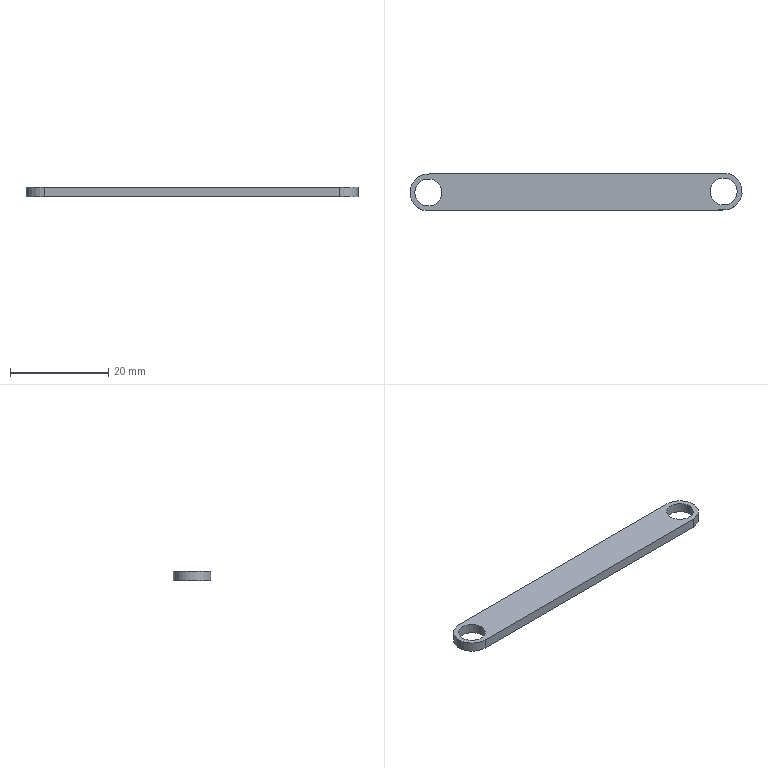Component | NX | CRANK_ROCKER_1 | 1 solid | 8 faces | box 67.5 x 7.69 x 2 mm | volume 893 mm3 | cylinder 4 | plane 4 | commonest cylinder face diameters 7.5 x2 5.5 x2
STEP:
#1=CARTESIAN_POINT('',(0.,0.,0.));
#2=DIRECTION('',(0.,0.,1.));
#3=DIRECTION('',(1.,0.,0.));
#4=AXIS2_PLACEMENT_3D('',#1,#2,#3);
#5=CARTESIAN_POINT('',(-30.015,-12.024,-10.49));
#6=VERTEX_POINT('',#5);
#7=CARTESIAN_POINT('',(-29.991,-19.524,-10.49));
#8=VERTEX_POINT('',#7);
#9=CARTESIAN_POINT('',(-30.003,-15.774,-10.49));
#10=DIRECTION('',(0.,0.,1.));
#11=DIRECTION('',(1.,0.003165,0.));
#12=AXIS2_PLACEMENT_3D('',#9,#10,#11);
#13=CIRCLE('',#12,3.75);
#14=CARTESIAN_POINT('',(-30.003,-15.774,-8.49));
#15=DIRECTION('',(0.,0.,-1.));
#16=DIRECTION('',(-1.,-0.003165,0.));
#17=AXIS2_PLACEMENT_3D('',#14,#15,#16);
#18=CYLINDRICAL_SURFACE('',#17,3.75);
#19=CARTESIAN_POINT('',(9.425,2.));
#20=DIRECTION('',(-1.,0.));
#21=VECTOR('',#20,1.);
#22=LINE('',#19,#21);
#23=(GEOMETRIC_REPRESENTATION_CONTEXT(2)PARAMETRIC_REPRESENTATION_CONTEXT()REPRESENTATION_CONTEXT('',''));
#24=DEFINITIONAL_REPRESENTATION('',(#22),#23);
#25=PCURVE('',#18,#24);
#26=CARTESIAN_POINT('',(-30.003,-15.774,-10.49));
#27=DIRECTION('',(0.,0.,1.));
#28=DIRECTION('',(1.,0.003165,0.));
#29=AXIS2_PLACEMENT_3D('',#26,#27,#28);
#30=PLANE('',#29);
#31=CARTESIAN_POINT('',(0.,0.));
#32=DIRECTION('',(1.,-0.));
#33=AXIS2_PLACEMENT_2D('',#31,#32);
#34=CIRCLE('',#33,3.75);
#35=(GEOMETRIC_REPRESENTATION_CONTEXT(2)PARAMETRIC_REPRESENTATION_CONTEXT()REPRESENTATION_CONTEXT('',''));
#36=DEFINITIONAL_REPRESENTATION('',(#34),#35);
#37=PCURVE('',#30,#36);
#38=SURFACE_CURVE('',#13,(#25,#37),.PCURVE_S1.);
#39=EDGE_CURVE('',#6,#8,#38,.T.);
#40=ORIENTED_EDGE('',*,*,#39,.T.);
#41=CARTESIAN_POINT('',(-29.991,-19.524,-8.49));
#42=VERTEX_POINT('',#41);
#43=CARTESIAN_POINT('',(-29.991,-19.524,-8.49));
#44=DIRECTION('',(0.,0.,-1.));
#45=VECTOR('',#44,1.);
#46=LINE('',#43,#45);
#47=CARTESIAN_POINT('',(4.712,0.));
#48=DIRECTION('',(0.,1.));
#49=VECTOR('',#48,1.);
#50=LINE('',#47,#49);
#51=(GEOMETRIC_REPRESENTATION_CONTEXT(2)PARAMETRIC_REPRESENTATION_CONTEXT()REPRESENTATION_CONTEXT('',''));
#52=DEFINITIONAL_REPRESENTATION('',(#50),#51);
#53=PCURVE('',#18,#52);
#54=CARTESIAN_POINT('',(-29.991,-19.524,-8.49));
#55=DIRECTION('',(-0.003165,1.,0.));
#56=DIRECTION('',(-1.,-0.003165,0.));
#57=AXIS2_PLACEMENT_3D('',#54,#55,#56);
#58=PLANE('',#57);
#59=CARTESIAN_POINT('',(-0.,0.));
#60=DIRECTION('',(0.,-1.));
#61=VECTOR('',#60,1.);
#62=LINE('',#59,#61);
#63=(GEOMETRIC_REPRESENTATION_CONTEXT(2)PARAMETRIC_REPRESENTATION_CONTEXT()REPRESENTATION_CONTEXT('',''));
#64=DEFINITIONAL_REPRESENTATION('',(#62),#63);
#65=PCURVE('',#58,#64);
#66=SURFACE_CURVE('',#46,(#53,#65),.PCURVE_S1.);
#67=EDGE_CURVE('',#42,#8,#66,.T.);
#68=ORIENTED_EDGE('',*,*,#67,.F.);
#69=CARTESIAN_POINT('',(-30.015,-12.024,-8.49));
#70=VERTEX_POINT('',#69);
#71=CARTESIAN_POINT('',(-30.003,-15.774,-8.49));
#72=DIRECTION('',(0.,0.,1.));
#73=DIRECTION('',(1.,0.003165,0.));
#74=AXIS2_PLACEMENT_3D('',#71,#72,#73);
#75=CIRCLE('',#74,3.75);
#76=CARTESIAN_POINT('',(9.425,0.));
#77=DIRECTION('',(-1.,0.));
#78=VECTOR('',#77,1.);
#79=LINE('',#76,#78);
#80=(GEOMETRIC_REPRESENTATION_CONTEXT(2)PARAMETRIC_REPRESENTATION_CONTEXT()REPRESENTATION_CONTEXT('',''));
#81=DEFINITIONAL_REPRESENTATION('',(#79),#80);
#82=PCURVE('',#18,#81);
#83=CARTESIAN_POINT('',(-30.003,-15.774,-8.49));
#84=DIRECTION('',(0.,0.,1.));
#85=DIRECTION('',(1.,0.003165,0.));
#86=AXIS2_PLACEMENT_3D('',#83,#84,#85);
#87=PLANE('',#86);
#88=CARTESIAN_POINT('',(0.,0.));
#89=DIRECTION('',(1.,-0.));
#90=AXIS2_PLACEMENT_2D('',#88,#89);
#91=CIRCLE('',#90,3.75);
#92=(GEOMETRIC_REPRESENTATION_CONTEXT(2)PARAMETRIC_REPRESENTATION_CONTEXT()REPRESENTATION_CONTEXT('',''));
#93=DEFINITIONAL_REPRESENTATION('',(#91),#92);
#94=PCURVE('',#87,#93);
#95=SURFACE_CURVE('',#75,(#82,#94),.PCURVE_S1.);
#96=EDGE_CURVE('',#70,#42,#95,.T.);
#97=ORIENTED_EDGE('',*,*,#96,.F.);
#98=CARTESIAN_POINT('',(-30.015,-12.024,-8.49));
#99=DIRECTION('',(0.,0.,-1.));
#100=VECTOR('',#99,1.);
#101=LINE('',#98,#100);
#102=CARTESIAN_POINT('',(7.854,0.));
#103=DIRECTION('',(0.,1.));
#104=VECTOR('',#103,1.);
#105=LINE('',#102,#104);
#106=(GEOMETRIC_REPRESENTATION_CONTEXT(2)PARAMETRIC_REPRESENTATION_CONTEXT()REPRESENTATION_CONTEXT('',''));
#107=DEFINITIONAL_REPRESENTATION('',(#105),#106);
#108=PCURVE('',#18,#107);
#109=CARTESIAN_POINT('',(29.985,-11.835,-8.49));
#110=DIRECTION('',(0.003165,-1.,0.));
#111=DIRECTION('',(0.,0.,-1.));
#112=AXIS2_PLACEMENT_3D('',#109,#110,#111);
#113=PLANE('',#112);
#114=CARTESIAN_POINT('',(0.,-60.));
#115=DIRECTION('',(1.,0.));
#116=VECTOR('',#115,1.);
#117=LINE('',#114,#116);
#118=(GEOMETRIC_REPRESENTATION_CONTEXT(2)PARAMETRIC_REPRESENTATION_CONTEXT()REPRESENTATION_CONTEXT('',''));
#119=DEFINITIONAL_REPRESENTATION('',(#117),#118);
#120=PCURVE('',#113,#119);
#121=SURFACE_CURVE('',#101,(#108,#120),.PCURVE_S1.);
#122=EDGE_CURVE('',#70,#6,#121,.T.);
#123=ORIENTED_EDGE('',*,*,#122,.T.);
#124=EDGE_LOOP('',(#40,#68,#97,#123));
#125=FACE_BOUND('',#124,.T.);
#126=ADVANCED_FACE('',(#125),#18,.T.);
#127=CARTESIAN_POINT('',(30.008,-19.335,-10.49));
#128=VERTEX_POINT('',#127);
#129=CARTESIAN_POINT('',(-29.991,-19.524,-10.49));
#130=DIRECTION('',(1.,0.003165,0.));
#131=VECTOR('',#130,1.);
#132=LINE('',#129,#131);
#133=CARTESIAN_POINT('',(0.,-2.));
#134=DIRECTION('',(-1.,0.));
#135=VECTOR('',#134,1.);
#136=LINE('',#133,#135);
#137=(GEOMETRIC_REPRESENTATION_CONTEXT(2)PARAMETRIC_REPRESENTATION_CONTEXT()REPRESENTATION_CONTEXT('',''));
#138=DEFINITIONAL_REPRESENTATION('',(#136),#137);
#139=PCURVE('',#58,#138);
#140=CARTESIAN_POINT('',(0.,-3.75));
#141=DIRECTION('',(1.,-0.));
#142=VECTOR('',#141,1.);
#143=LINE('',#140,#142);
#144=(GEOMETRIC_REPRESENTATION_CONTEXT(2)PARAMETRIC_REPRESENTATION_CONTEXT()REPRESENTATION_CONTEXT('',''));
#145=DEFINITIONAL_REPRESENTATION('',(#143),#144);
#146=PCURVE('',#30,#145);
#147=SURFACE_CURVE('',#132,(#139,#146),.PCURVE_S1.);
#148=EDGE_CURVE('',#8,#128,#147,.T.);
#149=ORIENTED_EDGE('',*,*,#148,.T.);
#150=CARTESIAN_POINT('',(30.008,-19.335,-8.49));
#151=VERTEX_POINT('',#150);
#152=CARTESIAN_POINT('',(30.008,-19.335,-8.49));
#153=DIRECTION('',(0.,0.,-1.));
#154=VECTOR('',#153,1.);
#155=LINE('',#152,#154);
#156=CARTESIAN_POINT('',(-60.,0.));
#157=DIRECTION('',(0.,-1.));
#158=VECTOR('',#157,1.);
#159=LINE('',#156,#158);
#160=(GEOMETRIC_REPRESENTATION_CONTEXT(2)PARAMETRIC_REPRESENTATION_CONTEXT()REPRESENTATION_CONTEXT('',''));
#161=DEFINITIONAL_REPRESENTATION('',(#159),#160);
#162=PCURVE('',#58,#161);
#163=CARTESIAN_POINT('',(29.996,-15.585,-8.49));
#164=DIRECTION('',(0.,0.,-1.));
#165=DIRECTION('',(-1.,-0.003165,0.));
#166=AXIS2_PLACEMENT_3D('',#163,#164,#165);
#167=CYLINDRICAL_SURFACE('',#166,3.75);
#168=CARTESIAN_POINT('',(4.712,0.));
#169=DIRECTION('',(0.,1.));
#170=VECTOR('',#169,1.);
#171=LINE('',#168,#170);
#172=(GEOMETRIC_REPRESENTATION_CONTEXT(2)PARAMETRIC_REPRESENTATION_CONTEXT()REPRESENTATION_CONTEXT('',''));
#173=DEFINITIONAL_REPRESENTATION('',(#171),#172);
#174=PCURVE('',#167,#173);
#175=SURFACE_CURVE('',#155,(#162,#174),.PCURVE_S1.);
#176=EDGE_CURVE('',#151,#128,#175,.T.);
#177=ORIENTED_EDGE('',*,*,#176,.F.);
#178=CARTESIAN_POINT('',(-29.991,-19.524,-8.49));
#179=DIRECTION('',(1.,0.003165,0.));
#180=VECTOR('',#179,1.);
#181=LINE('',#178,#180);
#182=CARTESIAN_POINT('',(0.,0.));
#183=DIRECTION('',(-1.,0.));
#184=VECTOR('',#183,1.);
#185=LINE('',#182,#184);
#186=(GEOMETRIC_REPRESENTATION_CONTEXT(2)PARAMETRIC_REPRESENTATION_CONTEXT()REPRESENTATION_CONTEXT('',''));
#187=DEFINITIONAL_REPRESENTATION('',(#185),#186);
#188=PCURVE('',#58,#187);
#189=CARTESIAN_POINT('',(0.,-3.75));
#190=DIRECTION('',(1.,-0.));
#191=VECTOR('',#190,1.);
#192=LINE('',#189,#191);
#193=(GEOMETRIC_REPRESENTATION_CONTEXT(2)PARAMETRIC_REPRESENTATION_CONTEXT()REPRESENTATION_CONTEXT('',''));
#194=DEFINITIONAL_REPRESENTATION('',(#192),#193);
#195=PCURVE('',#87,#194);
#196=SURFACE_CURVE('',#181,(#188,#195),.PCURVE_S1.);
#197=EDGE_CURVE('',#42,#151,#196,.T.);
#198=ORIENTED_EDGE('',*,*,#197,.F.);
#199=ORIENTED_EDGE('',*,*,#67,.T.);
#200=EDGE_LOOP('',(#149,#177,#198,#199));
#201=FACE_BOUND('',#200,.T.);
#202=ADVANCED_FACE('',(#201),#58,.F.);
#203=CARTESIAN_POINT('',(29.985,-11.835,-10.49));
#204=VERTEX_POINT('',#203);
#205=CARTESIAN_POINT('',(29.996,-15.585,-10.49));
#206=DIRECTION('',(0.,0.,1.));
#207=DIRECTION('',(1.,0.003165,0.));
#208=AXIS2_PLACEMENT_3D('',#205,#206,#207);
#209=CIRCLE('',#208,3.75);
#210=CARTESIAN_POINT('',(9.425,2.));
#211=DIRECTION('',(-1.,0.));
#212=VECTOR('',#211,1.);
#213=LINE('',#210,#212);
#214=(GEOMETRIC_REPRESENTATION_CONTEXT(2)PARAMETRIC_REPRESENTATION_CONTEXT()REPRESENTATION_CONTEXT('',''));
#215=DEFINITIONAL_REPRESENTATION('',(#213),#214);
#216=PCURVE('',#167,#215);
#217=CARTESIAN_POINT('',(60.,-0.));
#218=DIRECTION('',(1.,-0.));
#219=AXIS2_PLACEMENT_2D('',#217,#218);
#220=CIRCLE('',#219,3.75);
#221=(GEOMETRIC_REPRESENTATION_CONTEXT(2)PARAMETRIC_REPRESENTATION_CONTEXT()REPRESENTATION_CONTEXT('',''));
#222=DEFINITIONAL_REPRESENTATION('',(#220),#221);
#223=PCURVE('',#30,#222);
#224=SURFACE_CURVE('',#209,(#216,#223),.PCURVE_S1.);
#225=EDGE_CURVE('',#128,#204,#224,.T.);
#226=ORIENTED_EDGE('',*,*,#225,.T.);
#227=CARTESIAN_POINT('',(29.985,-11.835,-8.49));
#228=VERTEX_POINT('',#227);
#229=CARTESIAN_POINT('',(29.985,-11.835,-8.49));
#230=DIRECTION('',(0.,0.,-1.));
#231=VECTOR('',#230,1.);
#232=LINE('',#229,#231);
#233=CARTESIAN_POINT('',(1.571,0.));
#234=DIRECTION('',(0.,1.));
#235=VECTOR('',#234,1.);
#236=LINE('',#233,#235);
#237=(GEOMETRIC_REPRESENTATION_CONTEXT(2)PARAMETRIC_REPRESENTATION_CONTEXT()REPRESENTATION_CONTEXT('',''));
#238=DEFINITIONAL_REPRESENTATION('',(#236),#237);
#239=PCURVE('',#167,#238);
#240=CARTESIAN_POINT('',(0.,0.));
#241=DIRECTION('',(1.,0.));
#242=VECTOR('',#241,1.);
#243=LINE('',#240,#242);
#244=(GEOMETRIC_REPRESENTATION_CONTEXT(2)PARAMETRIC_REPRESENTATION_CONTEXT()REPRESENTATION_CONTEXT('',''));
#245=DEFINITIONAL_REPRESENTATION('',(#243),#244);
#246=PCURVE('',#113,#245);
#247=SURFACE_CURVE('',#232,(#239,#246),.PCURVE_S1.);
#248=EDGE_CURVE('',#228,#204,#247,.T.);
#249=ORIENTED_EDGE('',*,*,#248,.F.);
#250=CARTESIAN_POINT('',(29.996,-15.585,-8.49));
#251=DIRECTION('',(0.,0.,1.));
#252=DIRECTION('',(1.,0.003165,0.));
#253=AXIS2_PLACEMENT_3D('',#250,#251,#252);
#254=CIRCLE('',#253,3.75);
#255=CARTESIAN_POINT('',(9.425,0.));
#256=DIRECTION('',(-1.,0.));
#257=VECTOR('',#256,1.);
#258=LINE('',#255,#257);
#259=(GEOMETRIC_REPRESENTATION_CONTEXT(2)PARAMETRIC_REPRESENTATION_CONTEXT()REPRESENTATION_CONTEXT('',''));
#260=DEFINITIONAL_REPRESENTATION('',(#258),#259);
#261=PCURVE('',#167,#260);
#262=CARTESIAN_POINT('',(60.,-0.));
#263=DIRECTION('',(1.,-0.));
#264=AXIS2_PLACEMENT_2D('',#262,#263);
#265=CIRCLE('',#264,3.75);
#266=(GEOMETRIC_REPRESENTATION_CONTEXT(2)PARAMETRIC_REPRESENTATION_CONTEXT()REPRESENTATION_CONTEXT('',''));
#267=DEFINITIONAL_REPRESENTATION('',(#265),#266);
#268=PCURVE('',#87,#267);
#269=SURFACE_CURVE('',#254,(#261,#268),.PCURVE_S1.);
#270=EDGE_CURVE('',#151,#228,#269,.T.);
#271=ORIENTED_EDGE('',*,*,#270,.F.);
#272=ORIENTED_EDGE('',*,*,#176,.T.);
#273=EDGE_LOOP('',(#226,#249,#271,#272));
#274=FACE_BOUND('',#273,.T.);
#275=ADVANCED_FACE('',(#274),#167,.T.);
#276=CARTESIAN_POINT('',(-27.253,-15.766,-8.49));
#277=VERTEX_POINT('',#276);
#278=CARTESIAN_POINT('',(-30.003,-15.774,-8.49));
#279=DIRECTION('',(0.,0.,1.));
#280=DIRECTION('',(1.,0.003165,0.));
#281=AXIS2_PLACEMENT_3D('',#278,#279,#280);
#282=CIRCLE('',#281,2.75);
#283=CARTESIAN_POINT('',(-30.003,-15.774,-8.49));
#284=DIRECTION('',(0.,0.,-1.));
#285=DIRECTION('',(-1.,-0.003165,0.));
#286=AXIS2_PLACEMENT_3D('',#283,#284,#285);
#287=CYLINDRICAL_SURFACE('',#286,2.75);
#288=CARTESIAN_POINT('',(9.425,0.));
#289=DIRECTION('',(-1.,0.));
#290=VECTOR('',#289,1.);
#291=LINE('',#288,#290);
#292=(GEOMETRIC_REPRESENTATION_CONTEXT(2)PARAMETRIC_REPRESENTATION_CONTEXT()REPRESENTATION_CONTEXT('',''));
#293=DEFINITIONAL_REPRESENTATION('',(#291),#292);
#294=PCURVE('',#287,#293);
#295=CARTESIAN_POINT('',(0.,0.));
#296=DIRECTION('',(1.,0.));
#297=AXIS2_PLACEMENT_2D('',#295,#296);
#298=CIRCLE('',#297,2.75);
#299=(GEOMETRIC_REPRESENTATION_CONTEXT(2)PARAMETRIC_REPRESENTATION_CONTEXT()REPRESENTATION_CONTEXT('',''));
#300=DEFINITIONAL_REPRESENTATION('',(#298),#299);
#301=PCURVE('',#87,#300);
#302=SURFACE_CURVE('',#282,(#294,#301),.PCURVE_S1.);
#303=EDGE_CURVE('',#277,#277,#302,.T.);
#304=ORIENTED_EDGE('',*,*,#303,.F.);
#305=CARTESIAN_POINT('',(-27.253,-15.766,-10.49));
#306=VERTEX_POINT('',#305);
#307=CARTESIAN_POINT('',(-27.253,-15.766,-8.49));
#308=CARTESIAN_POINT('',(-27.253,-15.766,-10.49));
#309=B_SPLINE_CURVE_WITH_KNOTS('',1,(#307,#308),.UNSPECIFIED.,.F.,.F.,(2,2),(0.,2.),.PIECEWISE_BEZIER_KNOTS.);
#310=CARTESIAN_POINT('',(9.425,0.));
#311=DIRECTION('',(0.,1.));
#312=VECTOR('',#311,1.);
#313=LINE('',#310,#312);
#314=(GEOMETRIC_REPRESENTATION_CONTEXT(2)PARAMETRIC_REPRESENTATION_CONTEXT()REPRESENTATION_CONTEXT('',''));
#315=DEFINITIONAL_REPRESENTATION('',(#313),#314);
#316=PCURVE('',#287,#315);
#317=CARTESIAN_POINT('',(3.142,0.));
#318=DIRECTION('',(0.,1.));
#319=VECTOR('',#318,1.);
#320=LINE('',#317,#319);
#321=(GEOMETRIC_REPRESENTATION_CONTEXT(2)PARAMETRIC_REPRESENTATION_CONTEXT()REPRESENTATION_CONTEXT('',''));
#322=DEFINITIONAL_REPRESENTATION('',(#320),#321);
#323=PCURVE('',#287,#322);
#324=SEAM_CURVE('',#309,(#316,#323),.PCURVE_S1.);
#325=EDGE_CURVE('',#277,#306,#324,.T.);
#326=ORIENTED_EDGE('',*,*,#325,.T.);
#327=CARTESIAN_POINT('',(-30.003,-15.774,-10.49));
#328=DIRECTION('',(0.,0.,1.));
#329=DIRECTION('',(1.,0.003165,0.));
#330=AXIS2_PLACEMENT_3D('',#327,#328,#329);
#331=CIRCLE('',#330,2.75);
#332=CARTESIAN_POINT('',(9.425,2.));
#333=DIRECTION('',(-1.,0.));
#334=VECTOR('',#333,1.);
#335=LINE('',#332,#334);
#336=(GEOMETRIC_REPRESENTATION_CONTEXT(2)PARAMETRIC_REPRESENTATION_CONTEXT()REPRESENTATION_CONTEXT('',''));
#337=DEFINITIONAL_REPRESENTATION('',(#335),#336);
#338=PCURVE('',#287,#337);
#339=CARTESIAN_POINT('',(0.,0.));
#340=DIRECTION('',(1.,0.));
#341=AXIS2_PLACEMENT_2D('',#339,#340);
#342=CIRCLE('',#341,2.75);
#343=(GEOMETRIC_REPRESENTATION_CONTEXT(2)PARAMETRIC_REPRESENTATION_CONTEXT()REPRESENTATION_CONTEXT('',''));
#344=DEFINITIONAL_REPRESENTATION('',(#342),#343);
#345=PCURVE('',#30,#344);
#346=SURFACE_CURVE('',#331,(#338,#345),.PCURVE_S1.);
#347=EDGE_CURVE('',#306,#306,#346,.T.);
#348=ORIENTED_EDGE('',*,*,#347,.T.);
#349=ORIENTED_EDGE('',*,*,#325,.F.);
#350=EDGE_LOOP('',(#304,#326,#348,#349));
#351=FACE_BOUND('',#350,.F.);
#352=ADVANCED_FACE('',(#351),#287,.F.);
#353=CARTESIAN_POINT('',(29.985,-11.835,-10.49));
#354=DIRECTION('',(-1.,-0.003165,0.));
#355=VECTOR('',#354,1.);
#356=LINE('',#353,#355);
#357=CARTESIAN_POINT('',(2.,0.));
#358=DIRECTION('',(0.,-1.));
#359=VECTOR('',#358,1.);
#360=LINE('',#357,#359);
#361=(GEOMETRIC_REPRESENTATION_CONTEXT(2)PARAMETRIC_REPRESENTATION_CONTEXT()REPRESENTATION_CONTEXT('',''));
#362=DEFINITIONAL_REPRESENTATION('',(#360),#361);
#363=PCURVE('',#113,#362);
#364=CARTESIAN_POINT('',(60.,3.75));
#365=DIRECTION('',(-1.,0.));
#366=VECTOR('',#365,1.);
#367=LINE('',#364,#366);
#368=(GEOMETRIC_REPRESENTATION_CONTEXT(2)PARAMETRIC_REPRESENTATION_CONTEXT()REPRESENTATION_CONTEXT('',''));
#369=DEFINITIONAL_REPRESENTATION('',(#367),#368);
#370=PCURVE('',#30,#369);
#371=SURFACE_CURVE('',#356,(#363,#370),.PCURVE_S1.);
#372=EDGE_CURVE('',#204,#6,#371,.T.);
#373=ORIENTED_EDGE('',*,*,#372,.T.);
#374=ORIENTED_EDGE('',*,*,#122,.F.);
#375=CARTESIAN_POINT('',(29.985,-11.835,-8.49));
#376=DIRECTION('',(-1.,-0.003165,0.));
#377=VECTOR('',#376,1.);
#378=LINE('',#375,#377);
#379=CARTESIAN_POINT('',(0.,0.));
#380=DIRECTION('',(0.,-1.));
#381=VECTOR('',#380,1.);
#382=LINE('',#379,#381);
#383=(GEOMETRIC_REPRESENTATION_CONTEXT(2)PARAMETRIC_REPRESENTATION_CONTEXT()REPRESENTATION_CONTEXT('',''));
#384=DEFINITIONAL_REPRESENTATION('',(#382),#383);
#385=PCURVE('',#113,#384);
#386=CARTESIAN_POINT('',(60.,3.75));
#387=DIRECTION('',(-1.,0.));
#388=VECTOR('',#387,1.);
#389=LINE('',#386,#388);
#390=(GEOMETRIC_REPRESENTATION_CONTEXT(2)PARAMETRIC_REPRESENTATION_CONTEXT()REPRESENTATION_CONTEXT('',''));
#391=DEFINITIONAL_REPRESENTATION('',(#389),#390);
#392=PCURVE('',#87,#391);
#393=SURFACE_CURVE('',#378,(#385,#392),.PCURVE_S1.);
#394=EDGE_CURVE('',#228,#70,#393,.T.);
#395=ORIENTED_EDGE('',*,*,#394,.F.);
#396=ORIENTED_EDGE('',*,*,#248,.T.);
#397=EDGE_LOOP('',(#373,#374,#395,#396));
#398=FACE_BOUND('',#397,.T.);
#399=ADVANCED_FACE('',(#398),#113,.F.);
#400=CARTESIAN_POINT('',(32.746,-15.576,-8.49));
#401=VERTEX_POINT('',#400);
#402=CARTESIAN_POINT('',(29.996,-15.585,-8.49));
#403=DIRECTION('',(0.,0.,1.));
#404=DIRECTION('',(1.,0.003165,0.));
#405=AXIS2_PLACEMENT_3D('',#402,#403,#404);
#406=CIRCLE('',#405,2.75);
#407=CARTESIAN_POINT('',(29.996,-15.585,-8.49));
#408=DIRECTION('',(0.,0.,-1.));
#409=DIRECTION('',(-1.,-0.003165,0.));
#410=AXIS2_PLACEMENT_3D('',#407,#408,#409);
#411=CYLINDRICAL_SURFACE('',#410,2.75);
#412=CARTESIAN_POINT('',(9.425,0.));
#413=DIRECTION('',(-1.,0.));
#414=VECTOR('',#413,1.);
#415=LINE('',#412,#414);
#416=(GEOMETRIC_REPRESENTATION_CONTEXT(2)PARAMETRIC_REPRESENTATION_CONTEXT()REPRESENTATION_CONTEXT('',''));
#417=DEFINITIONAL_REPRESENTATION('',(#415),#416);
#418=PCURVE('',#411,#417);
#419=CARTESIAN_POINT('',(60.,-0.));
#420=DIRECTION('',(1.,0.));
#421=AXIS2_PLACEMENT_2D('',#419,#420);
#422=CIRCLE('',#421,2.75);
#423=(GEOMETRIC_REPRESENTATION_CONTEXT(2)PARAMETRIC_REPRESENTATION_CONTEXT()REPRESENTATION_CONTEXT('',''));
#424=DEFINITIONAL_REPRESENTATION('',(#422),#423);
#425=PCURVE('',#87,#424);
#426=SURFACE_CURVE('',#406,(#418,#425),.PCURVE_S1.);
#427=EDGE_CURVE('',#401,#401,#426,.T.);
#428=ORIENTED_EDGE('',*,*,#427,.F.);
#429=CARTESIAN_POINT('',(32.746,-15.576,-10.49));
#430=VERTEX_POINT('',#429);
#431=CARTESIAN_POINT('',(32.746,-15.576,-8.49));
#432=CARTESIAN_POINT('',(32.746,-15.576,-10.49));
#433=B_SPLINE_CURVE_WITH_KNOTS('',1,(#431,#432),.UNSPECIFIED.,.F.,.F.,(2,2),(0.,2.),.PIECEWISE_BEZIER_KNOTS.);
#434=CARTESIAN_POINT('',(9.425,0.));
#435=DIRECTION('',(0.,1.));
#436=VECTOR('',#435,1.);
#437=LINE('',#434,#436);
#438=(GEOMETRIC_REPRESENTATION_CONTEXT(2)PARAMETRIC_REPRESENTATION_CONTEXT()REPRESENTATION_CONTEXT('',''));
#439=DEFINITIONAL_REPRESENTATION('',(#437),#438);
#440=PCURVE('',#411,#439);
#441=CARTESIAN_POINT('',(3.142,0.));
#442=DIRECTION('',(0.,1.));
#443=VECTOR('',#442,1.);
#444=LINE('',#441,#443);
#445=(GEOMETRIC_REPRESENTATION_CONTEXT(2)PARAMETRIC_REPRESENTATION_CONTEXT()REPRESENTATION_CONTEXT('',''));
#446=DEFINITIONAL_REPRESENTATION('',(#444),#445);
#447=PCURVE('',#411,#446);
#448=SEAM_CURVE('',#433,(#440,#447),.PCURVE_S1.);
#449=EDGE_CURVE('',#401,#430,#448,.T.);
#450=ORIENTED_EDGE('',*,*,#449,.T.);
#451=CARTESIAN_POINT('',(29.996,-15.585,-10.49));
#452=DIRECTION('',(0.,0.,1.));
#453=DIRECTION('',(1.,0.003165,0.));
#454=AXIS2_PLACEMENT_3D('',#451,#452,#453);
#455=CIRCLE('',#454,2.75);
#456=CARTESIAN_POINT('',(9.425,2.));
#457=DIRECTION('',(-1.,0.));
#458=VECTOR('',#457,1.);
#459=LINE('',#456,#458);
#460=(GEOMETRIC_REPRESENTATION_CONTEXT(2)PARAMETRIC_REPRESENTATION_CONTEXT()REPRESENTATION_CONTEXT('',''));
#461=DEFINITIONAL_REPRESENTATION('',(#459),#460);
#462=PCURVE('',#411,#461);
#463=CARTESIAN_POINT('',(60.,-0.));
#464=DIRECTION('',(1.,0.));
#465=AXIS2_PLACEMENT_2D('',#463,#464);
#466=CIRCLE('',#465,2.75);
#467=(GEOMETRIC_REPRESENTATION_CONTEXT(2)PARAMETRIC_REPRESENTATION_CONTEXT()REPRESENTATION_CONTEXT('',''));
#468=DEFINITIONAL_REPRESENTATION('',(#466),#467);
#469=PCURVE('',#30,#468);
#470=SURFACE_CURVE('',#455,(#462,#469),.PCURVE_S1.);
#471=EDGE_CURVE('',#430,#430,#470,.T.);
#472=ORIENTED_EDGE('',*,*,#471,.T.);
#473=ORIENTED_EDGE('',*,*,#449,.F.);
#474=EDGE_LOOP('',(#428,#450,#472,#473));
#475=FACE_BOUND('',#474,.F.);
#476=ADVANCED_FACE('',(#475),#411,.F.);
#477=ORIENTED_EDGE('',*,*,#96,.T.);
#478=ORIENTED_EDGE('',*,*,#197,.T.);
#479=ORIENTED_EDGE('',*,*,#270,.T.);
#480=ORIENTED_EDGE('',*,*,#394,.T.);
#481=EDGE_LOOP('',(#477,#478,#479,#480));
#482=FACE_BOUND('',#481,.T.);
#483=ORIENTED_EDGE('',*,*,#303,.F.);
#484=EDGE_LOOP('',(#483));
#485=FACE_BOUND('',#484,.T.);
#486=ORIENTED_EDGE('',*,*,#427,.F.);
#487=EDGE_LOOP('',(#486));
#488=FACE_BOUND('',#487,.T.);
#489=ADVANCED_FACE('',(#482,#485,#488),#87,.T.);
#490=ORIENTED_EDGE('',*,*,#39,.F.);
#491=ORIENTED_EDGE('',*,*,#372,.F.);
#492=ORIENTED_EDGE('',*,*,#225,.F.);
#493=ORIENTED_EDGE('',*,*,#148,.F.);
#494=EDGE_LOOP('',(#490,#491,#492,#493));
#495=FACE_BOUND('',#494,.T.);
#496=ORIENTED_EDGE('',*,*,#347,.T.);
#497=EDGE_LOOP('',(#496));
#498=FACE_BOUND('',#497,.T.);
#499=ORIENTED_EDGE('',*,*,#471,.T.);
#500=EDGE_LOOP('',(#499));
#501=FACE_BOUND('',#500,.T.);
#502=ADVANCED_FACE('',(#495,#498,#501),#30,.F.);
#503=CLOSED_SHELL('',(#126,#202,#275,#352,#399,#476,#489,#502));
#504=MANIFOLD_SOLID_BREP('',#503);
#505=(LENGTH_UNIT()NAMED_UNIT(*)SI_UNIT(.MILLI.,.METRE.));
#506=UNCERTAINTY_MEASURE_WITH_UNIT(LENGTH_MEASURE(0.000002),#505,'','');
#507=(NAMED_UNIT(*)PLANE_ANGLE_UNIT()SI_UNIT($,.RADIAN.));
#508=(NAMED_UNIT(*)SI_UNIT($,.STERADIAN.)SOLID_ANGLE_UNIT());
#509=(GEOMETRIC_REPRESENTATION_CONTEXT(3)GLOBAL_UNCERTAINTY_ASSIGNED_CONTEXT((#506))GLOBAL_UNIT_ASSIGNED_CONTEXT((#505,#507,#508))REPRESENTATION_CONTEXT('',''));
#510=ADVANCED_BREP_SHAPE_REPRESENTATION('',(#4,#504),#509);